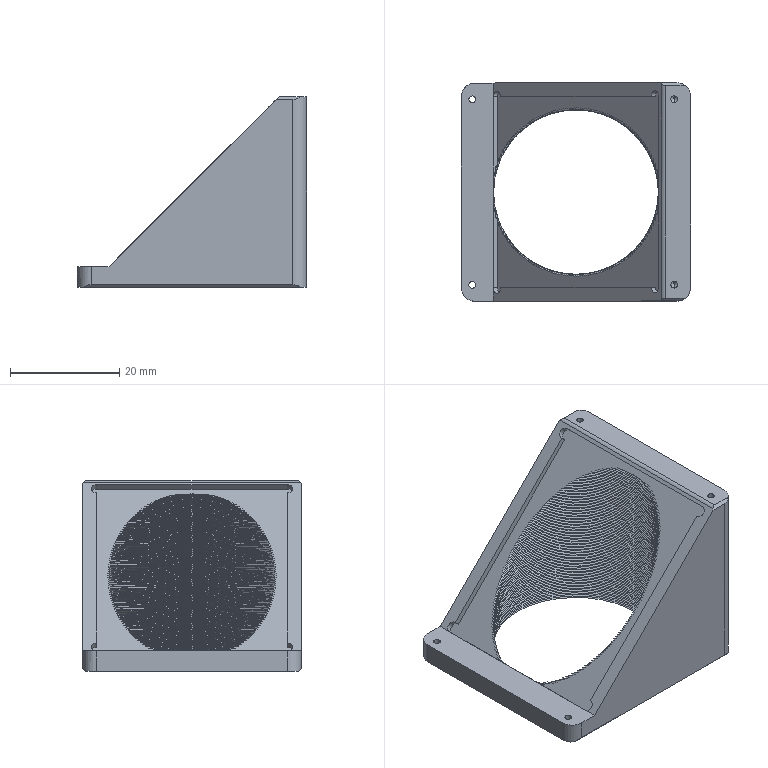CAM job | Mastercam | mm | 27 operations | part box 42 x 40 x 35
1. Facing | 24 - 80 平铣刀
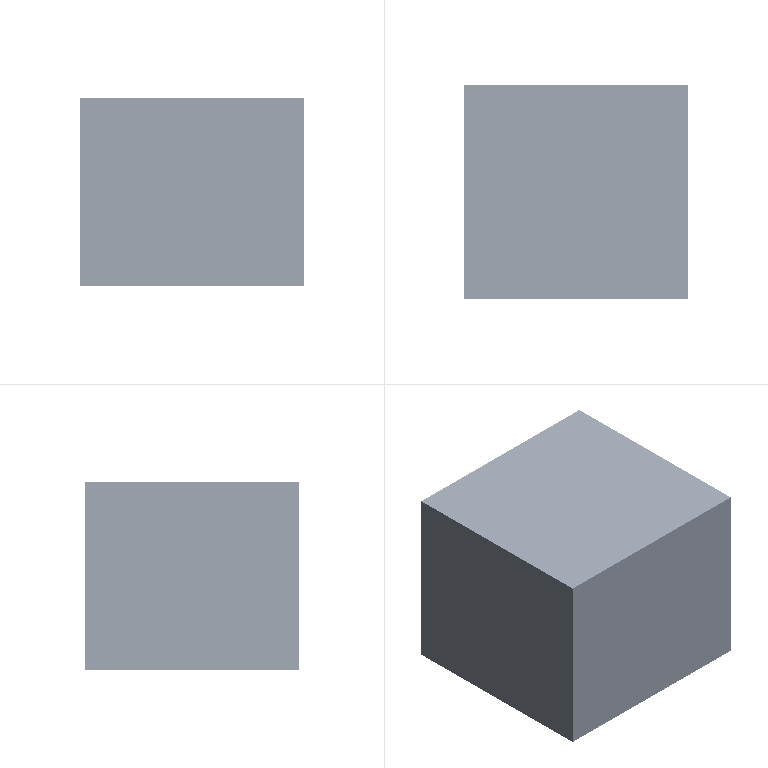2. Drill/Counterbore | 1 - 6 倒角刀
3. Peck Drill | 20 - 1.25 钻头
4. 3D High Speed (Dynamic OptiRough) | 8 - 8C
5. Contour (2D) | 9 - 8J
6. Contour (2D) | 9 - 8J
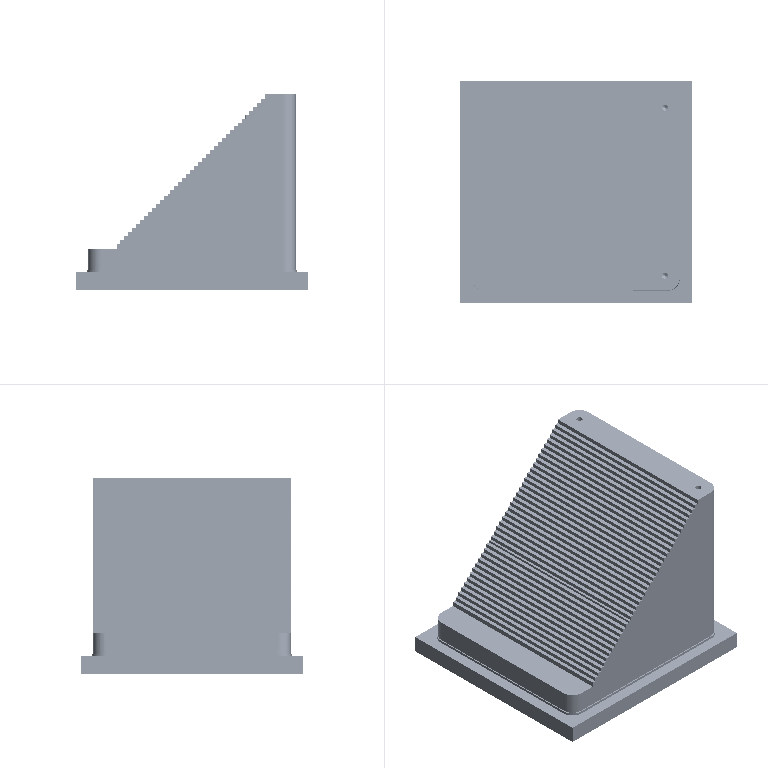7. Contour (2D chamfer) | 1 - 6 倒角刀
8. Surface Finish Flowline | 17 - 4 圆鼻铣刀
9. Facing | 24 - 80 平铣刀
10. Facing | 24 - 80 平铣刀
11. 3D High Speed (Dynamic OptiRough) | 8 - 8C
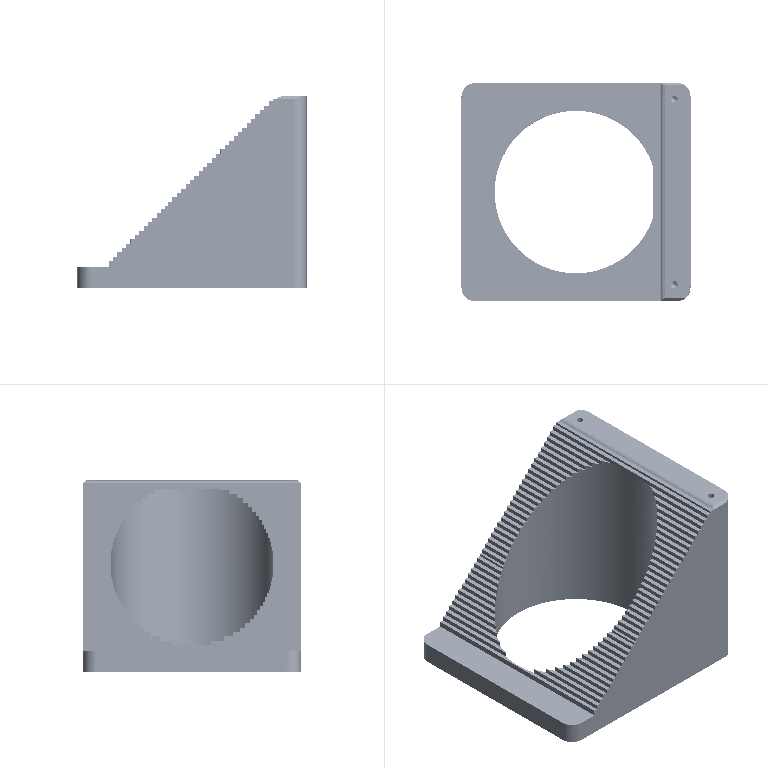12. Contour (2D) | 9 - 8J
13. Contour (Remachining) | 4 - 4C
14. Contour (2D) | 5 - 4J
15. Contour (Remachining) | 3 - 2J
16. Drill/Counterbore | 1 - 6 倒角刀
17. Peck Drill | 20 - 1.25 钻头
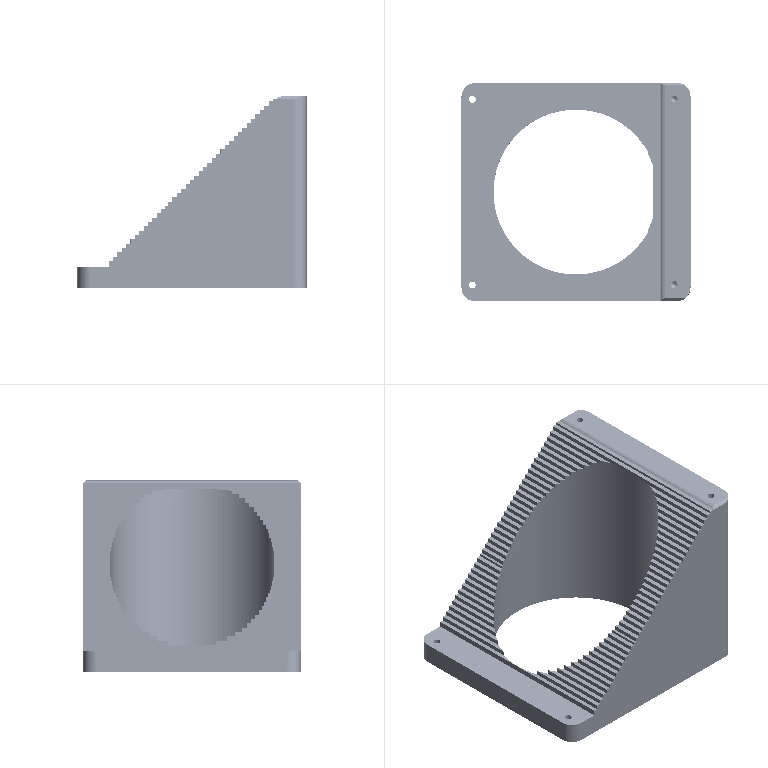18. Contour (2D chamfer) | 1 - 6 倒角刀
19. Contour (2D chamfer) | 1 - 6 倒角刀
20. Chamfer Drill | 1 - 6 倒角刀
21. Contour (2D) | 2 - 4.75 螺纹铣刀
22. Contour (2D) | 9 - 8J
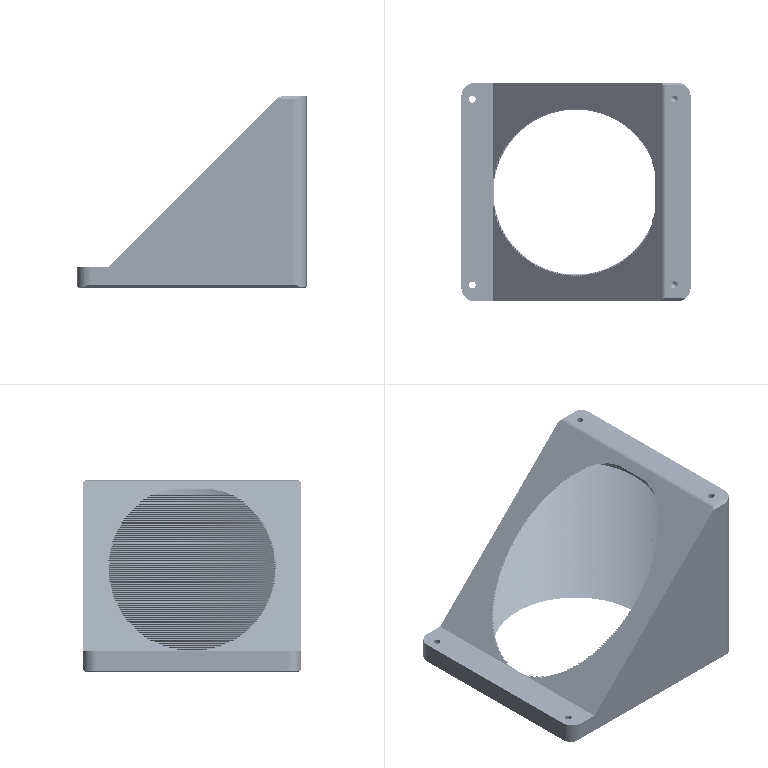23. 2D High Speed (2D Dynamic Mill) | 8 - 8C
24. Contour (Remachining) | 4 - 4C
25. 2D High Speed (2D Area Mill) | 5 - 4J
26. Contour (2D) | 5 - 4J
27. Contour (Remachining) | 3 - 2J